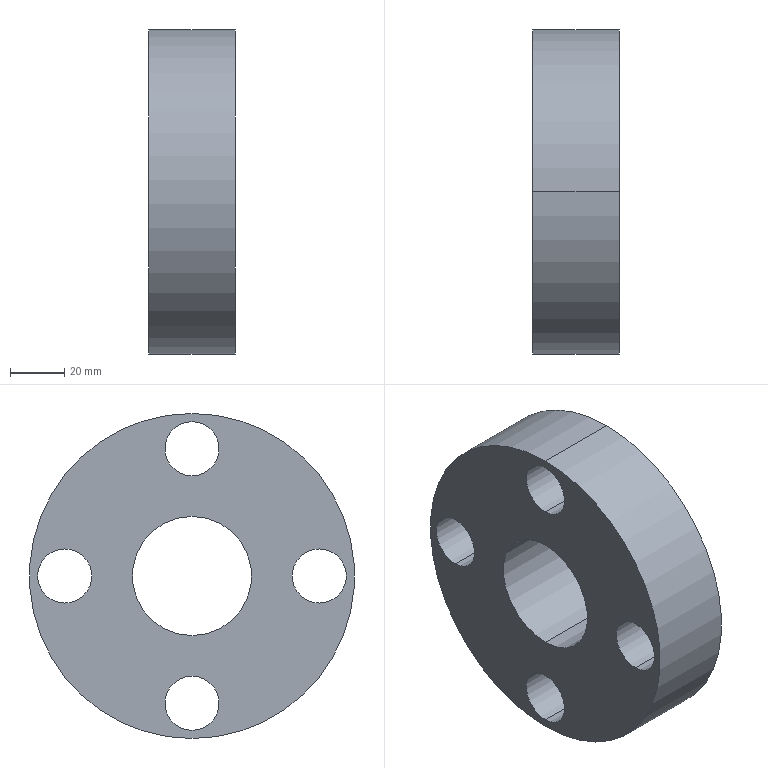Component | SolidWorks | RotatingDisk-1 | 1 solid | 14 faces | box 32 x 120 x 120 mm | volume 273042 mm3 | cylinder 12 | plane 2 | commonest cylinder face diameters 20 x8 44 x2 120 x2
build123d program:
from build123d import *

# Parameters (mm, degrees)
SKETCH1_R           = 60
SKETCH1_R_2         = 10
SKETCH1_R_3         = 22
BOSS_EXTRUDE1_DEPTH = 32


with BuildPart() as part:
    # Sketch1 → Boss-Extrude1 (new body)
    with BuildSketch(Plane(origin=(0, 0, 0), x_dir=(0, 0, -1), z_dir=(1, 0, 0))):
        Circle(SKETCH1_R)
        with Locations((0, 47)):
            Circle(SKETCH1_R_2, mode=Mode.SUBTRACT)
        with Locations((47, 0)):
            Circle(SKETCH1_R_2, mode=Mode.SUBTRACT)
        with Locations((0, -47)):
            Circle(SKETCH1_R_2, mode=Mode.SUBTRACT)
        with Locations((-47, 0)):
            Circle(SKETCH1_R_2, mode=Mode.SUBTRACT)
        Circle(SKETCH1_R_3, mode=Mode.SUBTRACT)
    extrude(amount=BOSS_EXTRUDE1_DEPTH)


solid = part.part

# Placed as in the assembly
solid = solid.moved(Location((496.528, 15.31, -240), (0, 0, 0)))
STEP:
#1=COLOUR_RGB('',0.7922,0.8196,0.9333);
#2=FILL_AREA_STYLE_COLOUR('',#1);
#3=FILL_AREA_STYLE('',(#2));
#4=SURFACE_STYLE_FILL_AREA(#3);
#5=SURFACE_SIDE_STYLE('',(#4));
#6=SURFACE_STYLE_USAGE(.BOTH.,#5);
#7=PRESENTATION_STYLE_ASSIGNMENT((#6));
#8=CARTESIAN_POINT('',(20.808,0.6028,-7.205));
#9=VERTEX_POINT('',#8);
#10=CARTESIAN_POINT('',(20.808,0.6028,-7.992));
#11=VERTEX_POINT('',#10);
#12=CARTESIAN_POINT('',(20.808,0.6028,-7.598));
#13=DIRECTION('',(1.,0.,0.));
#14=DIRECTION('',(0.,0.,-1.));
#15=AXIS2_PLACEMENT_3D('',#12,#13,#14);
#16=CIRCLE('',#15,0.3937);
#17=EDGE_CURVE('',#9,#11,#16,.T.);
#18=ORIENTED_EDGE('',*,*,#17,.T.);
#19=CARTESIAN_POINT('',(19.548,0.6028,-7.992));
#20=VERTEX_POINT('',#19);
#21=CARTESIAN_POINT('',(20.808,0.6028,-7.992));
#22=DIRECTION('',(-1.,0.,0.));
#23=VECTOR('',#22,39.37);
#24=LINE('',#21,#23);
#25=EDGE_CURVE('',#11,#20,#24,.T.);
#26=ORIENTED_EDGE('',*,*,#25,.T.);
#27=CARTESIAN_POINT('',(19.548,0.6028,-7.205));
#28=VERTEX_POINT('',#27);
#29=CARTESIAN_POINT('',(19.548,0.6028,-7.598));
#30=DIRECTION('',(1.,0.,0.));
#31=DIRECTION('',(0.,0.,-1.));
#32=AXIS2_PLACEMENT_3D('',#29,#30,#31);
#33=CIRCLE('',#32,0.3937);
#34=EDGE_CURVE('',#28,#20,#33,.T.);
#35=ORIENTED_EDGE('',*,*,#34,.F.);
#36=CARTESIAN_POINT('',(20.808,0.6028,-7.205));
#37=DIRECTION('',(-1.,0.,0.));
#38=VECTOR('',#37,39.37);
#39=LINE('',#36,#38);
#40=EDGE_CURVE('',#9,#28,#39,.T.);
#41=ORIENTED_EDGE('',*,*,#40,.F.);
#42=EDGE_LOOP('',(#18,#26,#35,#41));
#43=FACE_OUTER_BOUND('',#42,.T.);
#44=CARTESIAN_POINT('',(20.808,0.6028,-7.598));
#45=DIRECTION('',(-1.,0.,0.));
#46=DIRECTION('',(0.,0.,1.));
#47=AXIS2_PLACEMENT_3D('',#44,#45,#46);
#48=CYLINDRICAL_SURFACE('',#47,0.3937);
#49=ADVANCED_FACE('',(#43),#48,.F.);
#50=CARTESIAN_POINT('',(20.808,-1.248,-9.055));
#51=VERTEX_POINT('',#50);
#52=CARTESIAN_POINT('',(20.808,-1.248,-9.843));
#53=VERTEX_POINT('',#52);
#54=CARTESIAN_POINT('',(20.808,-1.248,-9.449));
#55=DIRECTION('',(1.,0.,0.));
#56=DIRECTION('',(0.,0.,-1.));
#57=AXIS2_PLACEMENT_3D('',#54,#55,#56);
#58=CIRCLE('',#57,0.3937);
#59=EDGE_CURVE('',#51,#53,#58,.T.);
#60=ORIENTED_EDGE('',*,*,#59,.T.);
#61=CARTESIAN_POINT('',(19.548,-1.248,-9.843));
#62=VERTEX_POINT('',#61);
#63=CARTESIAN_POINT('',(20.808,-1.248,-9.843));
#64=DIRECTION('',(-1.,0.,0.));
#65=VECTOR('',#64,39.37);
#66=LINE('',#63,#65);
#67=EDGE_CURVE('',#53,#62,#66,.T.);
#68=ORIENTED_EDGE('',*,*,#67,.T.);
#69=CARTESIAN_POINT('',(19.548,-1.248,-9.055));
#70=VERTEX_POINT('',#69);
#71=CARTESIAN_POINT('',(19.548,-1.248,-9.449));
#72=DIRECTION('',(1.,0.,0.));
#73=DIRECTION('',(0.,0.,-1.));
#74=AXIS2_PLACEMENT_3D('',#71,#72,#73);
#75=CIRCLE('',#74,0.3937);
#76=EDGE_CURVE('',#70,#62,#75,.T.);
#77=ORIENTED_EDGE('',*,*,#76,.F.);
#78=CARTESIAN_POINT('',(20.808,-1.248,-9.055));
#79=DIRECTION('',(-1.,0.,0.));
#80=VECTOR('',#79,39.37);
#81=LINE('',#78,#80);
#82=EDGE_CURVE('',#51,#70,#81,.T.);
#83=ORIENTED_EDGE('',*,*,#82,.F.);
#84=EDGE_LOOP('',(#60,#68,#77,#83));
#85=FACE_OUTER_BOUND('',#84,.T.);
#86=CARTESIAN_POINT('',(20.808,-1.248,-9.449));
#87=DIRECTION('',(-1.,0.,0.));
#88=DIRECTION('',(0.,0.,1.));
#89=AXIS2_PLACEMENT_3D('',#86,#87,#88);
#90=CYLINDRICAL_SURFACE('',#89,0.3937);
#91=ADVANCED_FACE('',(#85),#90,.F.);
#92=CARTESIAN_POINT('',(20.808,0.6028,-10.906));
#93=VERTEX_POINT('',#92);
#94=CARTESIAN_POINT('',(20.808,0.6028,-11.693));
#95=VERTEX_POINT('',#94);
#96=CARTESIAN_POINT('',(20.808,0.6028,-11.299));
#97=DIRECTION('',(1.,0.,0.));
#98=DIRECTION('',(0.,0.,-1.));
#99=AXIS2_PLACEMENT_3D('',#96,#97,#98);
#100=CIRCLE('',#99,0.3937);
#101=EDGE_CURVE('',#93,#95,#100,.T.);
#102=ORIENTED_EDGE('',*,*,#101,.T.);
#103=CARTESIAN_POINT('',(19.548,0.6028,-11.693));
#104=VERTEX_POINT('',#103);
#105=CARTESIAN_POINT('',(20.808,0.6028,-11.693));
#106=DIRECTION('',(-1.,0.,0.));
#107=VECTOR('',#106,39.37);
#108=LINE('',#105,#107);
#109=EDGE_CURVE('',#95,#104,#108,.T.);
#110=ORIENTED_EDGE('',*,*,#109,.T.);
#111=CARTESIAN_POINT('',(19.548,0.6028,-10.906));
#112=VERTEX_POINT('',#111);
#113=CARTESIAN_POINT('',(19.548,0.6028,-11.299));
#114=DIRECTION('',(1.,0.,0.));
#115=DIRECTION('',(0.,0.,-1.));
#116=AXIS2_PLACEMENT_3D('',#113,#114,#115);
#117=CIRCLE('',#116,0.3937);
#118=EDGE_CURVE('',#112,#104,#117,.T.);
#119=ORIENTED_EDGE('',*,*,#118,.F.);
#120=CARTESIAN_POINT('',(20.808,0.6028,-10.906));
#121=DIRECTION('',(-1.,0.,0.));
#122=VECTOR('',#121,39.37);
#123=LINE('',#120,#122);
#124=EDGE_CURVE('',#93,#112,#123,.T.);
#125=ORIENTED_EDGE('',*,*,#124,.F.);
#126=EDGE_LOOP('',(#102,#110,#119,#125));
#127=FACE_OUTER_BOUND('',#126,.T.);
#128=CARTESIAN_POINT('',(20.808,0.6028,-11.299));
#129=DIRECTION('',(-1.,0.,0.));
#130=DIRECTION('',(0.,0.,1.));
#131=AXIS2_PLACEMENT_3D('',#128,#129,#130);
#132=CYLINDRICAL_SURFACE('',#131,0.3937);
#133=ADVANCED_FACE('',(#127),#132,.F.);
#134=CARTESIAN_POINT('',(20.808,0.6028,-8.583));
#135=VERTEX_POINT('',#134);
#136=CARTESIAN_POINT('',(20.808,0.6028,-10.315));
#137=VERTEX_POINT('',#136);
#138=CARTESIAN_POINT('',(20.808,0.6028,-9.449));
#139=DIRECTION('',(1.,0.,0.));
#140=DIRECTION('',(0.,0.,-1.));
#141=AXIS2_PLACEMENT_3D('',#138,#139,#140);
#142=CIRCLE('',#141,0.8661);
#143=EDGE_CURVE('',#135,#137,#142,.T.);
#144=ORIENTED_EDGE('',*,*,#143,.T.);
#145=CARTESIAN_POINT('',(19.548,0.6028,-10.315));
#146=VERTEX_POINT('',#145);
#147=CARTESIAN_POINT('',(20.808,0.6028,-10.315));
#148=DIRECTION('',(-1.,0.,0.));
#149=VECTOR('',#148,39.37);
#150=LINE('',#147,#149);
#151=EDGE_CURVE('',#137,#146,#150,.T.);
#152=ORIENTED_EDGE('',*,*,#151,.T.);
#153=CARTESIAN_POINT('',(19.548,0.6028,-8.583));
#154=VERTEX_POINT('',#153);
#155=CARTESIAN_POINT('',(19.548,0.6028,-9.449));
#156=DIRECTION('',(1.,0.,0.));
#157=DIRECTION('',(0.,0.,-1.));
#158=AXIS2_PLACEMENT_3D('',#155,#156,#157);
#159=CIRCLE('',#158,0.8661);
#160=EDGE_CURVE('',#154,#146,#159,.T.);
#161=ORIENTED_EDGE('',*,*,#160,.F.);
#162=CARTESIAN_POINT('',(20.808,0.6028,-8.583));
#163=DIRECTION('',(-1.,0.,0.));
#164=VECTOR('',#163,39.37);
#165=LINE('',#162,#164);
#166=EDGE_CURVE('',#135,#154,#165,.T.);
#167=ORIENTED_EDGE('',*,*,#166,.F.);
#168=EDGE_LOOP('',(#144,#152,#161,#167));
#169=FACE_OUTER_BOUND('',#168,.T.);
#170=CARTESIAN_POINT('',(20.808,0.6028,-9.449));
#171=DIRECTION('',(-1.,0.,0.));
#172=DIRECTION('',(0.,0.,1.));
#173=AXIS2_PLACEMENT_3D('',#170,#171,#172);
#174=CYLINDRICAL_SURFACE('',#173,0.8661);
#175=ADVANCED_FACE('',(#169),#174,.F.);
#176=CARTESIAN_POINT('',(20.808,2.453,-9.055));
#177=VERTEX_POINT('',#176);
#178=CARTESIAN_POINT('',(20.808,2.453,-9.843));
#179=VERTEX_POINT('',#178);
#180=CARTESIAN_POINT('',(20.808,2.453,-9.449));
#181=DIRECTION('',(1.,0.,0.));
#182=DIRECTION('',(0.,0.,-1.));
#183=AXIS2_PLACEMENT_3D('',#180,#181,#182);
#184=CIRCLE('',#183,0.3937);
#185=EDGE_CURVE('',#177,#179,#184,.T.);
#186=ORIENTED_EDGE('',*,*,#185,.T.);
#187=CARTESIAN_POINT('',(19.548,2.453,-9.843));
#188=VERTEX_POINT('',#187);
#189=CARTESIAN_POINT('',(20.808,2.453,-9.843));
#190=DIRECTION('',(-1.,0.,0.));
#191=VECTOR('',#190,39.37);
#192=LINE('',#189,#191);
#193=EDGE_CURVE('',#179,#188,#192,.T.);
#194=ORIENTED_EDGE('',*,*,#193,.T.);
#195=CARTESIAN_POINT('',(19.548,2.453,-9.055));
#196=VERTEX_POINT('',#195);
#197=CARTESIAN_POINT('',(19.548,2.453,-9.449));
#198=DIRECTION('',(1.,0.,0.));
#199=DIRECTION('',(0.,0.,-1.));
#200=AXIS2_PLACEMENT_3D('',#197,#198,#199);
#201=CIRCLE('',#200,0.3937);
#202=EDGE_CURVE('',#196,#188,#201,.T.);
#203=ORIENTED_EDGE('',*,*,#202,.F.);
#204=CARTESIAN_POINT('',(20.808,2.453,-9.055));
#205=DIRECTION('',(-1.,0.,0.));
#206=VECTOR('',#205,39.37);
#207=LINE('',#204,#206);
#208=EDGE_CURVE('',#177,#196,#207,.T.);
#209=ORIENTED_EDGE('',*,*,#208,.F.);
#210=EDGE_LOOP('',(#186,#194,#203,#209));
#211=FACE_OUTER_BOUND('',#210,.T.);
#212=CARTESIAN_POINT('',(20.808,2.453,-9.449));
#213=DIRECTION('',(-1.,0.,0.));
#214=DIRECTION('',(0.,0.,1.));
#215=AXIS2_PLACEMENT_3D('',#212,#213,#214);
#216=CYLINDRICAL_SURFACE('',#215,0.3937);
#217=ADVANCED_FACE('',(#211),#216,.F.);
#218=CARTESIAN_POINT('',(20.808,0.6028,-11.811));
#219=VERTEX_POINT('',#218);
#220=CARTESIAN_POINT('',(20.808,0.6028,-7.087));
#221=VERTEX_POINT('',#220);
#222=CARTESIAN_POINT('',(20.808,0.6028,-9.449));
#223=DIRECTION('',(1.,0.,0.));
#224=DIRECTION('',(0.,0.,-1.));
#225=AXIS2_PLACEMENT_3D('',#222,#223,#224);
#226=CIRCLE('',#225,2.362);
#227=EDGE_CURVE('',#219,#221,#226,.T.);
#228=ORIENTED_EDGE('',*,*,#227,.F.);
#229=CARTESIAN_POINT('',(19.548,0.6028,-11.811));
#230=VERTEX_POINT('',#229);
#231=CARTESIAN_POINT('',(20.808,0.6028,-11.811));
#232=DIRECTION('',(-1.,0.,0.));
#233=VECTOR('',#232,39.37);
#234=LINE('',#231,#233);
#235=EDGE_CURVE('',#219,#230,#234,.T.);
#236=ORIENTED_EDGE('',*,*,#235,.T.);
#237=CARTESIAN_POINT('',(19.548,0.6028,-7.087));
#238=VERTEX_POINT('',#237);
#239=CARTESIAN_POINT('',(19.548,0.6028,-9.449));
#240=DIRECTION('',(1.,0.,0.));
#241=DIRECTION('',(0.,0.,-1.));
#242=AXIS2_PLACEMENT_3D('',#239,#240,#241);
#243=CIRCLE('',#242,2.362);
#244=EDGE_CURVE('',#230,#238,#243,.T.);
#245=ORIENTED_EDGE('',*,*,#244,.T.);
#246=CARTESIAN_POINT('',(20.808,0.6028,-7.087));
#247=DIRECTION('',(-1.,0.,0.));
#248=VECTOR('',#247,39.37);
#249=LINE('',#246,#248);
#250=EDGE_CURVE('',#221,#238,#249,.T.);
#251=ORIENTED_EDGE('',*,*,#250,.F.);
#252=EDGE_LOOP('',(#228,#236,#245,#251));
#253=FACE_OUTER_BOUND('',#252,.T.);
#254=CARTESIAN_POINT('',(20.808,0.6028,-9.449));
#255=DIRECTION('',(-1.,0.,0.));
#256=DIRECTION('',(0.,0.,1.));
#257=AXIS2_PLACEMENT_3D('',#254,#255,#256);
#258=CYLINDRICAL_SURFACE('',#257,2.362);
#259=ADVANCED_FACE('',(#253),#258,.T.);
#260=ORIENTED_EDGE('',*,*,#59,.F.);
#261=CARTESIAN_POINT('',(20.808,-1.248,-9.449));
#262=DIRECTION('',(1.,0.,0.));
#263=DIRECTION('',(0.,0.,-1.));
#264=AXIS2_PLACEMENT_3D('',#261,#262,#263);
#265=CIRCLE('',#264,0.3937);
#266=EDGE_CURVE('',#53,#51,#265,.T.);
#267=ORIENTED_EDGE('',*,*,#266,.F.);
#268=EDGE_LOOP('',(#260,#267));
#269=FACE_BOUND('',#268,.T.);
#270=ORIENTED_EDGE('',*,*,#143,.F.);
#271=CARTESIAN_POINT('',(20.808,0.6028,-9.449));
#272=DIRECTION('',(1.,0.,0.));
#273=DIRECTION('',(0.,0.,-1.));
#274=AXIS2_PLACEMENT_3D('',#271,#272,#273);
#275=CIRCLE('',#274,0.8661);
#276=EDGE_CURVE('',#137,#135,#275,.T.);
#277=ORIENTED_EDGE('',*,*,#276,.F.);
#278=EDGE_LOOP('',(#270,#277));
#279=FACE_BOUND('',#278,.T.);
#280=CARTESIAN_POINT('',(20.808,0.6028,-9.449));
#281=DIRECTION('',(1.,0.,0.));
#282=DIRECTION('',(0.,0.,-1.));
#283=AXIS2_PLACEMENT_3D('',#280,#281,#282);
#284=CIRCLE('',#283,2.362);
#285=EDGE_CURVE('',#221,#219,#284,.T.);
#286=ORIENTED_EDGE('',*,*,#285,.T.);
#287=ORIENTED_EDGE('',*,*,#227,.T.);
#288=EDGE_LOOP('',(#286,#287));
#289=FACE_OUTER_BOUND('',#288,.T.);
#290=ORIENTED_EDGE('',*,*,#185,.F.);
#291=CARTESIAN_POINT('',(20.808,2.453,-9.449));
#292=DIRECTION('',(1.,0.,0.));
#293=DIRECTION('',(0.,0.,-1.));
#294=AXIS2_PLACEMENT_3D('',#291,#292,#293);
#295=CIRCLE('',#294,0.3937);
#296=EDGE_CURVE('',#179,#177,#295,.T.);
#297=ORIENTED_EDGE('',*,*,#296,.F.);
#298=EDGE_LOOP('',(#290,#297));
#299=FACE_BOUND('',#298,.T.);
#300=ORIENTED_EDGE('',*,*,#101,.F.);
#301=CARTESIAN_POINT('',(20.808,0.6028,-11.299));
#302=DIRECTION('',(1.,0.,0.));
#303=DIRECTION('',(0.,0.,-1.));
#304=AXIS2_PLACEMENT_3D('',#301,#302,#303);
#305=CIRCLE('',#304,0.3937);
#306=EDGE_CURVE('',#95,#93,#305,.T.);
#307=ORIENTED_EDGE('',*,*,#306,.F.);
#308=EDGE_LOOP('',(#300,#307));
#309=FACE_BOUND('',#308,.T.);
#310=ORIENTED_EDGE('',*,*,#17,.F.);
#311=CARTESIAN_POINT('',(20.808,0.6028,-7.598));
#312=DIRECTION('',(1.,0.,0.));
#313=DIRECTION('',(0.,0.,-1.));
#314=AXIS2_PLACEMENT_3D('',#311,#312,#313);
#315=CIRCLE('',#314,0.3937);
#316=EDGE_CURVE('',#11,#9,#315,.T.);
#317=ORIENTED_EDGE('',*,*,#316,.F.);
#318=EDGE_LOOP('',(#310,#317));
#319=FACE_BOUND('',#318,.T.);
#320=CARTESIAN_POINT('',(20.808,0.6028,-9.449));
#321=DIRECTION('',(1.,0.,0.));
#322=DIRECTION('',(0.,0.,-1.));
#323=AXIS2_PLACEMENT_3D('',#320,#321,#322);
#324=PLANE('',#323);
#325=ADVANCED_FACE('',(#269,#279,#289,#299,#309,#319),#324,.T.);
#326=CARTESIAN_POINT('',(19.548,0.6028,-9.449));
#327=DIRECTION('',(1.,0.,0.));
#328=DIRECTION('',(0.,0.,-1.));
#329=AXIS2_PLACEMENT_3D('',#326,#327,#328);
#330=CIRCLE('',#329,2.362);
#331=EDGE_CURVE('',#238,#230,#330,.T.);
#332=ORIENTED_EDGE('',*,*,#331,.F.);
#333=ORIENTED_EDGE('',*,*,#244,.F.);
#334=EDGE_LOOP('',(#332,#333));
#335=FACE_OUTER_BOUND('',#334,.T.);
#336=ORIENTED_EDGE('',*,*,#202,.T.);
#337=CARTESIAN_POINT('',(19.548,2.453,-9.449));
#338=DIRECTION('',(1.,0.,0.));
#339=DIRECTION('',(0.,0.,-1.));
#340=AXIS2_PLACEMENT_3D('',#337,#338,#339);
#341=CIRCLE('',#340,0.3937);
#342=EDGE_CURVE('',#188,#196,#341,.T.);
#343=ORIENTED_EDGE('',*,*,#342,.T.);
#344=EDGE_LOOP('',(#336,#343));
#345=FACE_BOUND('',#344,.T.);
#346=ORIENTED_EDGE('',*,*,#160,.T.);
#347=CARTESIAN_POINT('',(19.548,0.6028,-9.449));
#348=DIRECTION('',(1.,0.,0.));
#349=DIRECTION('',(0.,0.,-1.));
#350=AXIS2_PLACEMENT_3D('',#347,#348,#349);
#351=CIRCLE('',#350,0.8661);
#352=EDGE_CURVE('',#146,#154,#351,.T.);
#353=ORIENTED_EDGE('',*,*,#352,.T.);
#354=EDGE_LOOP('',(#346,#353));
#355=FACE_BOUND('',#354,.T.);
#356=ORIENTED_EDGE('',*,*,#118,.T.);
#357=CARTESIAN_POINT('',(19.548,0.6028,-11.299));
#358=DIRECTION('',(1.,0.,0.));
#359=DIRECTION('',(0.,0.,-1.));
#360=AXIS2_PLACEMENT_3D('',#357,#358,#359);
#361=CIRCLE('',#360,0.3937);
#362=EDGE_CURVE('',#104,#112,#361,.T.);
#363=ORIENTED_EDGE('',*,*,#362,.T.);
#364=EDGE_LOOP('',(#356,#363));
#365=FACE_BOUND('',#364,.T.);
#366=ORIENTED_EDGE('',*,*,#76,.T.);
#367=CARTESIAN_POINT('',(19.548,-1.248,-9.449));
#368=DIRECTION('',(1.,0.,0.));
#369=DIRECTION('',(0.,0.,-1.));
#370=AXIS2_PLACEMENT_3D('',#367,#368,#369);
#371=CIRCLE('',#370,0.3937);
#372=EDGE_CURVE('',#62,#70,#371,.T.);
#373=ORIENTED_EDGE('',*,*,#372,.T.);
#374=EDGE_LOOP('',(#366,#373));
#375=FACE_BOUND('',#374,.T.);
#376=ORIENTED_EDGE('',*,*,#34,.T.);
#377=CARTESIAN_POINT('',(19.548,0.6028,-7.598));
#378=DIRECTION('',(1.,0.,0.));
#379=DIRECTION('',(0.,0.,-1.));
#380=AXIS2_PLACEMENT_3D('',#377,#378,#379);
#381=CIRCLE('',#380,0.3937);
#382=EDGE_CURVE('',#20,#28,#381,.T.);
#383=ORIENTED_EDGE('',*,*,#382,.T.);
#384=EDGE_LOOP('',(#376,#383));
#385=FACE_BOUND('',#384,.T.);
#386=CARTESIAN_POINT('',(19.548,0.6028,-9.449));
#387=DIRECTION('',(1.,0.,0.));
#388=DIRECTION('',(0.,0.,-1.));
#389=AXIS2_PLACEMENT_3D('',#386,#387,#388);
#390=PLANE('',#389);
#391=ADVANCED_FACE('',(#335,#345,#355,#365,#375,#385),#390,.F.);
#392=ORIENTED_EDGE('',*,*,#235,.F.);
#393=ORIENTED_EDGE('',*,*,#285,.F.);
#394=ORIENTED_EDGE('',*,*,#250,.T.);
#395=ORIENTED_EDGE('',*,*,#331,.T.);
#396=EDGE_LOOP('',(#392,#393,#394,#395));
#397=FACE_OUTER_BOUND('',#396,.T.);
#398=CARTESIAN_POINT('',(20.808,0.6028,-9.449));
#399=DIRECTION('',(-1.,0.,0.));
#400=DIRECTION('',(0.,0.,1.));
#401=AXIS2_PLACEMENT_3D('',#398,#399,#400);
#402=CYLINDRICAL_SURFACE('',#401,2.362);
#403=ADVANCED_FACE('',(#397),#402,.T.);
#404=ORIENTED_EDGE('',*,*,#193,.F.);
#405=ORIENTED_EDGE('',*,*,#296,.T.);
#406=ORIENTED_EDGE('',*,*,#208,.T.);
#407=ORIENTED_EDGE('',*,*,#342,.F.);
#408=EDGE_LOOP('',(#404,#405,#406,#407));
#409=FACE_OUTER_BOUND('',#408,.T.);
#410=CARTESIAN_POINT('',(20.808,2.453,-9.449));
#411=DIRECTION('',(-1.,0.,0.));
#412=DIRECTION('',(0.,0.,1.));
#413=AXIS2_PLACEMENT_3D('',#410,#411,#412);
#414=CYLINDRICAL_SURFACE('',#413,0.3937);
#415=ADVANCED_FACE('',(#409),#414,.F.);
#416=ORIENTED_EDGE('',*,*,#151,.F.);
#417=ORIENTED_EDGE('',*,*,#276,.T.);
#418=ORIENTED_EDGE('',*,*,#166,.T.);
#419=ORIENTED_EDGE('',*,*,#352,.F.);
#420=EDGE_LOOP('',(#416,#417,#418,#419));
#421=FACE_OUTER_BOUND('',#420,.T.);
#422=CARTESIAN_POINT('',(20.808,0.6028,-9.449));
#423=DIRECTION('',(-1.,0.,0.));
#424=DIRECTION('',(0.,0.,1.));
#425=AXIS2_PLACEMENT_3D('',#422,#423,#424);
#426=CYLINDRICAL_SURFACE('',#425,0.8661);
#427=ADVANCED_FACE('',(#421),#426,.F.);
#428=ORIENTED_EDGE('',*,*,#109,.F.);
#429=ORIENTED_EDGE('',*,*,#306,.T.);
#430=ORIENTED_EDGE('',*,*,#124,.T.);
#431=ORIENTED_EDGE('',*,*,#362,.F.);
#432=EDGE_LOOP('',(#428,#429,#430,#431));
#433=FACE_OUTER_BOUND('',#432,.T.);
#434=CARTESIAN_POINT('',(20.808,0.6028,-11.299));
#435=DIRECTION('',(-1.,0.,0.));
#436=DIRECTION('',(0.,0.,1.));
#437=AXIS2_PLACEMENT_3D('',#434,#435,#436);
#438=CYLINDRICAL_SURFACE('',#437,0.3937);
#439=ADVANCED_FACE('',(#433),#438,.F.);
#440=ORIENTED_EDGE('',*,*,#67,.F.);
#441=ORIENTED_EDGE('',*,*,#266,.T.);
#442=ORIENTED_EDGE('',*,*,#82,.T.);
#443=ORIENTED_EDGE('',*,*,#372,.F.);
#444=EDGE_LOOP('',(#440,#441,#442,#443));
#445=FACE_OUTER_BOUND('',#444,.T.);
#446=CARTESIAN_POINT('',(20.808,-1.248,-9.449));
#447=DIRECTION('',(-1.,0.,0.));
#448=DIRECTION('',(0.,0.,1.));
#449=AXIS2_PLACEMENT_3D('',#446,#447,#448);
#450=CYLINDRICAL_SURFACE('',#449,0.3937);
#451=ADVANCED_FACE('',(#445),#450,.F.);
#452=ORIENTED_EDGE('',*,*,#25,.F.);
#453=ORIENTED_EDGE('',*,*,#316,.T.);
#454=ORIENTED_EDGE('',*,*,#40,.T.);
#455=ORIENTED_EDGE('',*,*,#382,.F.);
#456=EDGE_LOOP('',(#452,#453,#454,#455));
#457=FACE_OUTER_BOUND('',#456,.T.);
#458=CARTESIAN_POINT('',(20.808,0.6028,-7.598));
#459=DIRECTION('',(-1.,0.,0.));
#460=DIRECTION('',(0.,0.,1.));
#461=AXIS2_PLACEMENT_3D('',#458,#459,#460);
#462=CYLINDRICAL_SURFACE('',#461,0.3937);
#463=ADVANCED_FACE('',(#457),#462,.F.);
#464=CLOSED_SHELL('',(#49,#91,#133,#175,#217,#259,#325,#391,#403,#415,#427,#439,#451,#463));
#465=MANIFOLD_SOLID_BREP('',#464);
#466=STYLED_ITEM('',(#7),#465);
#467=(LENGTH_UNIT()NAMED_UNIT(*)SI_UNIT($,.METRE.));
#468=LENGTH_MEASURE_WITH_UNIT(LENGTH_MEASURE(0.0254),#467);
#469=DIMENSIONAL_EXPONENTS(1.,0.,0.,0.,0.,0.,0.);
#470=(CONVERSION_BASED_UNIT('',#468)LENGTH_UNIT()NAMED_UNIT(#469));
#471=UNCERTAINTY_MEASURE_WITH_UNIT(LENGTH_MEASURE(0.00001),#470,'','');
#472=(NAMED_UNIT(*)PLANE_ANGLE_UNIT()SI_UNIT($,.RADIAN.));
#473=(NAMED_UNIT(*)SI_UNIT($,.STERADIAN.)SOLID_ANGLE_UNIT());
#474=(GEOMETRIC_REPRESENTATION_CONTEXT(3)GLOBAL_UNCERTAINTY_ASSIGNED_CONTEXT((#471))GLOBAL_UNIT_ASSIGNED_CONTEXT((#470,#472,#473))REPRESENTATION_CONTEXT('',''));
#475=MECHANICAL_DESIGN_GEOMETRIC_PRESENTATION_REPRESENTATION('',(#466),#474);
#476=CARTESIAN_POINT('',(0.,0.,0.));
#477=DIRECTION('',(0.,0.,1.));
#478=DIRECTION('',(1.,0.,0.));
#479=AXIS2_PLACEMENT_3D('',#476,#477,#478);
#480=(LENGTH_UNIT()NAMED_UNIT(*)SI_UNIT($,.METRE.));
#481=LENGTH_MEASURE_WITH_UNIT(LENGTH_MEASURE(0.0254),#480);
#482=DIMENSIONAL_EXPONENTS(1.,0.,0.,0.,0.,0.,0.);
#483=(CONVERSION_BASED_UNIT('',#481)LENGTH_UNIT()NAMED_UNIT(#482));
#484=UNCERTAINTY_MEASURE_WITH_UNIT(LENGTH_MEASURE(0.00001),#483,'','');
#485=(NAMED_UNIT(*)PLANE_ANGLE_UNIT()SI_UNIT($,.RADIAN.));
#486=(NAMED_UNIT(*)SI_UNIT($,.STERADIAN.)SOLID_ANGLE_UNIT());
#487=(GEOMETRIC_REPRESENTATION_CONTEXT(3)GLOBAL_UNCERTAINTY_ASSIGNED_CONTEXT((#484))GLOBAL_UNIT_ASSIGNED_CONTEXT((#483,#485,#486))REPRESENTATION_CONTEXT('',''));
#488=ADVANCED_BREP_SHAPE_REPRESENTATION('',(#465,#479),#487);
#489=PRESENTATION_LAYER_ASSIGNMENT('','',(#466));